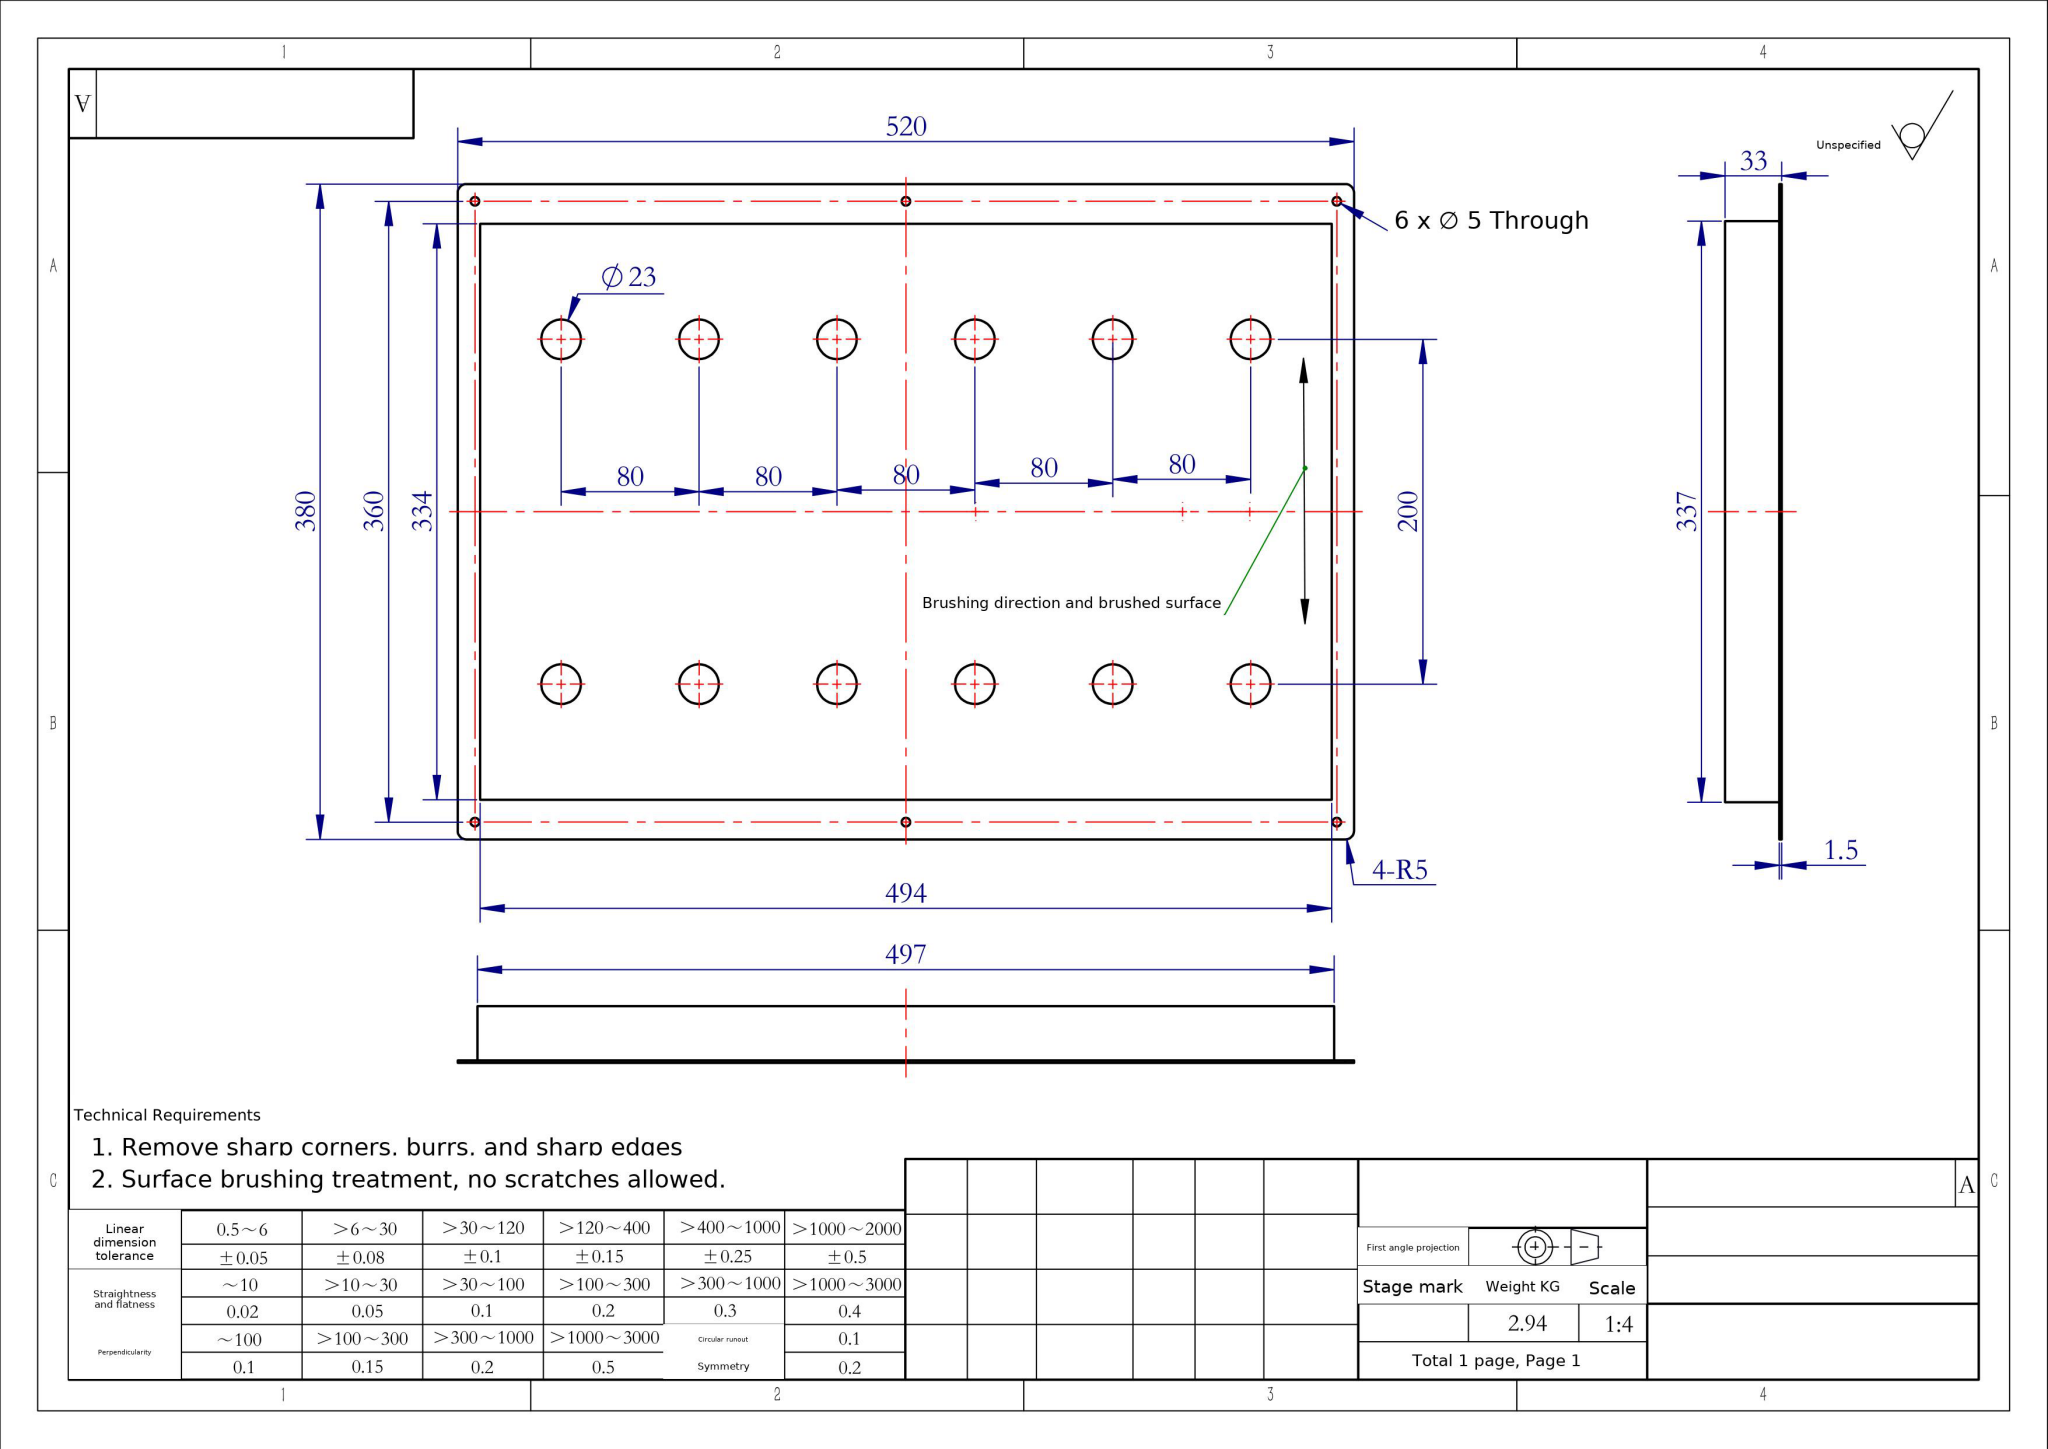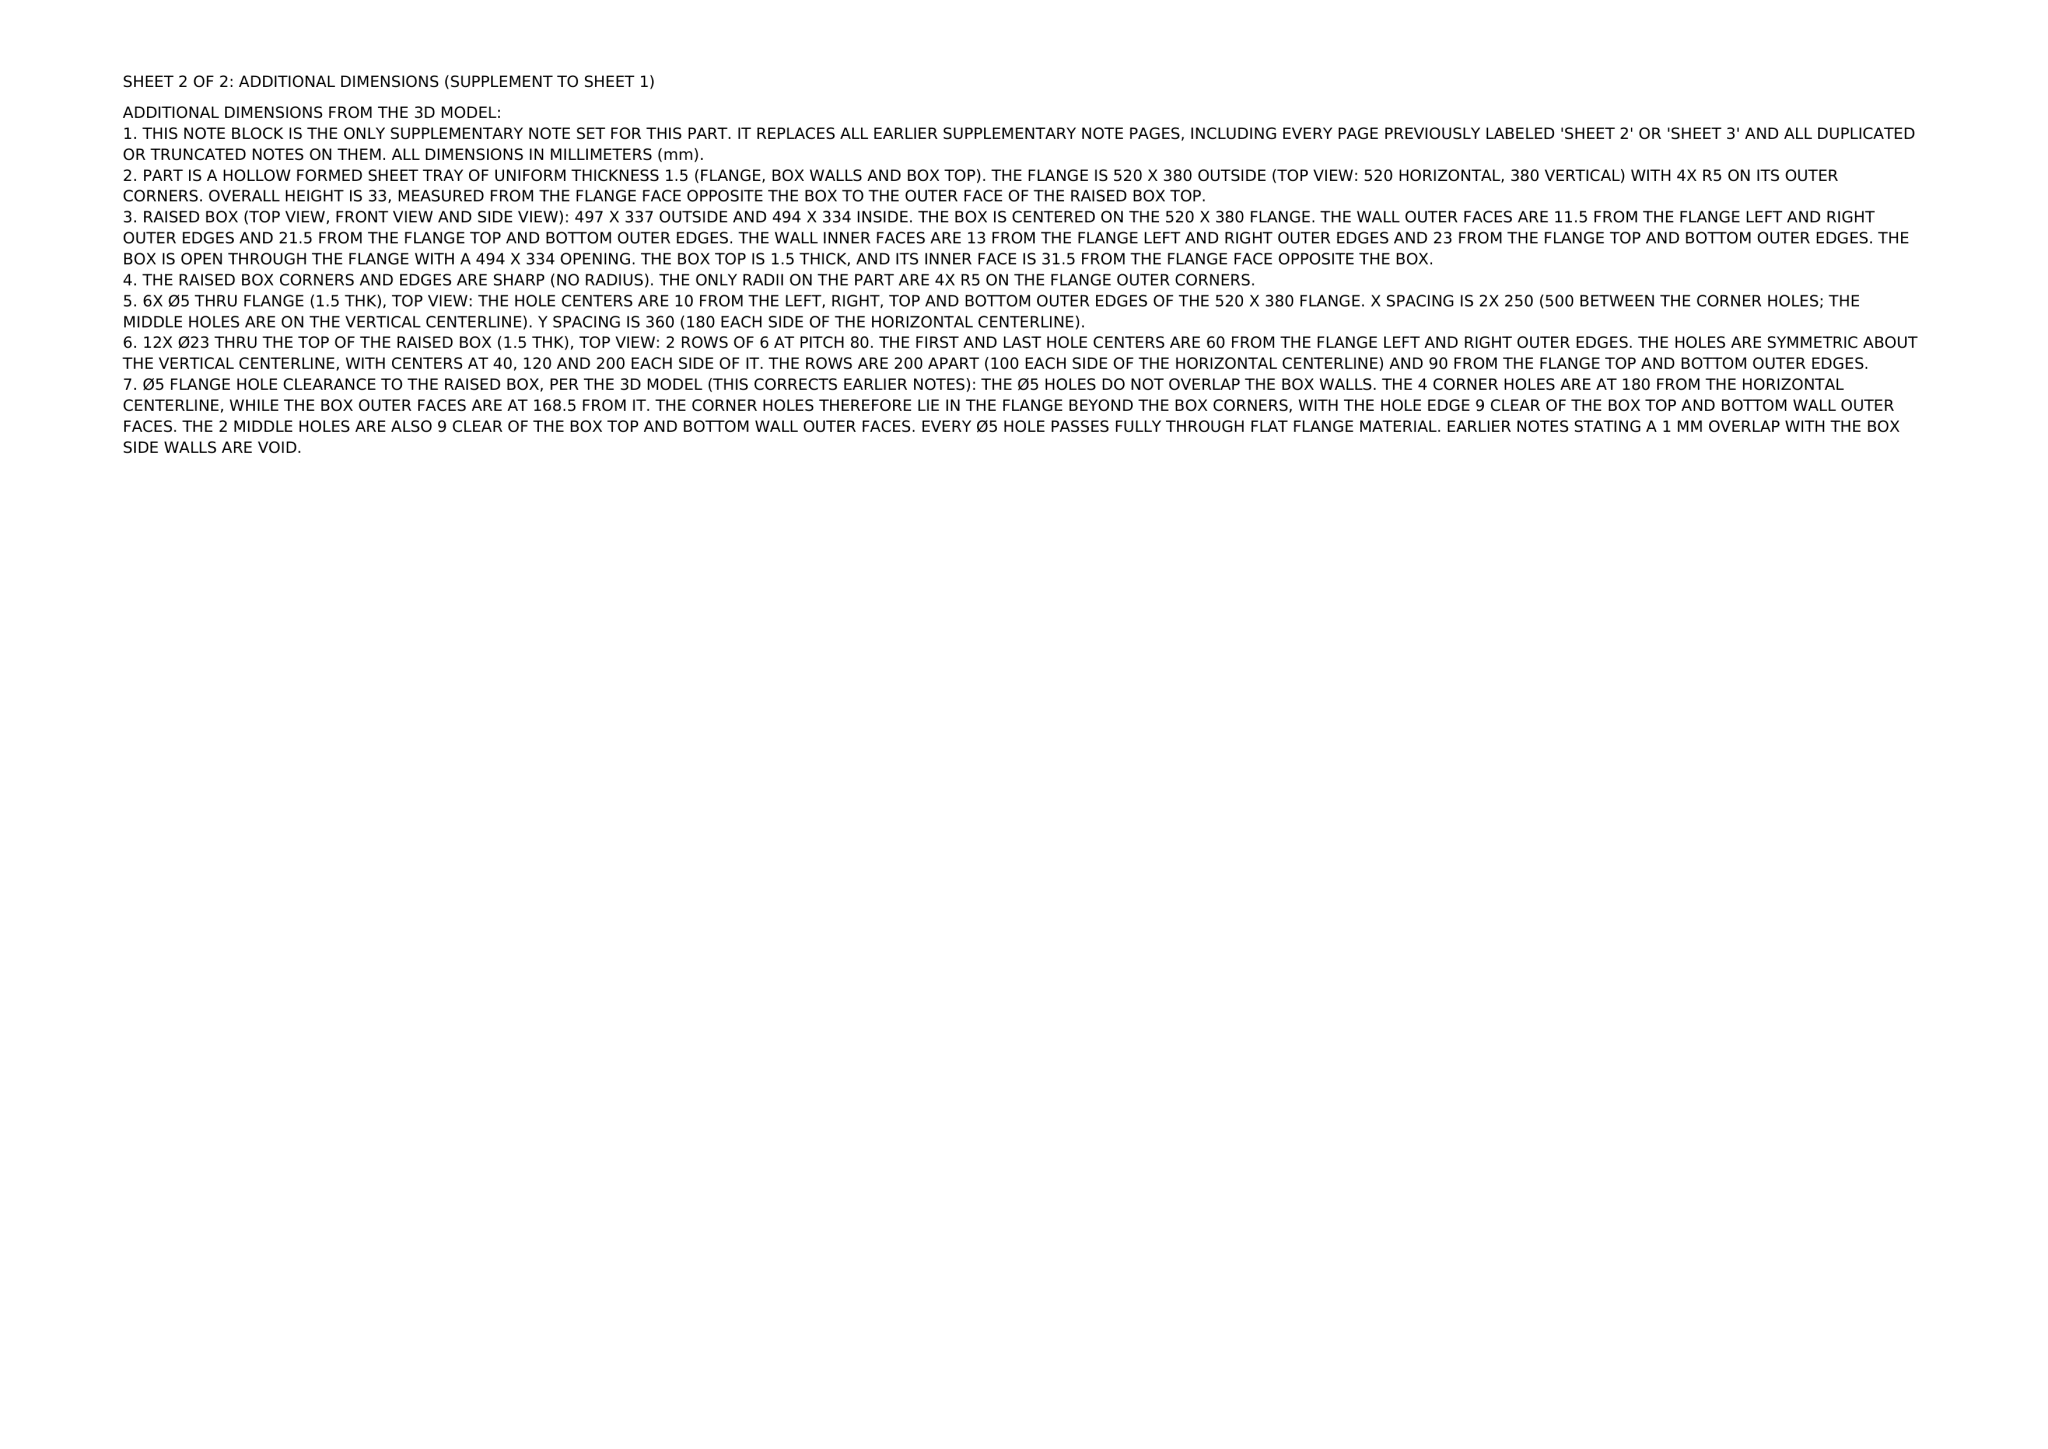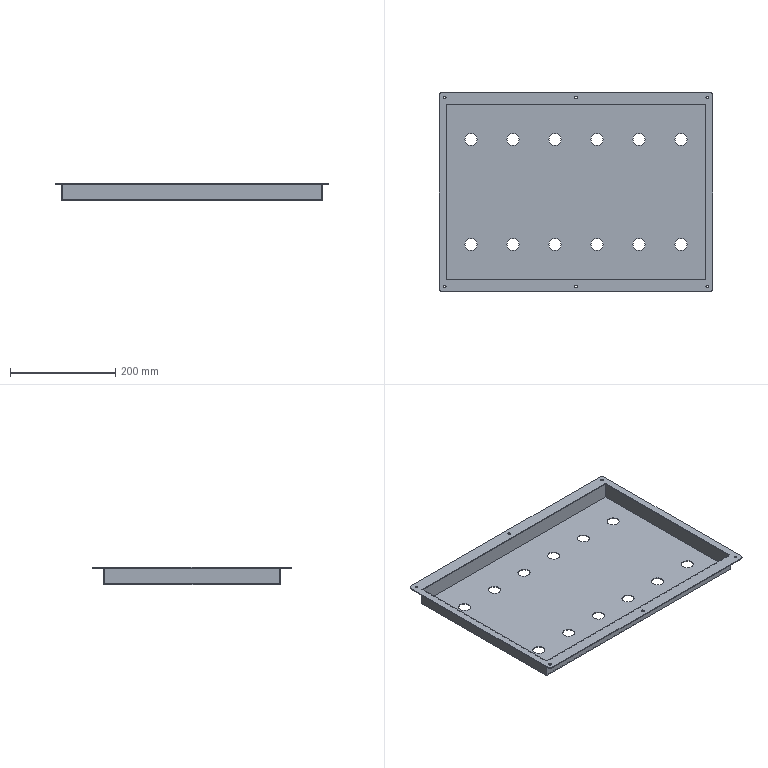Part | NX | mm | 1 solid | 60 faces | box 520 x 380 x 33 mm | volume 367242 mm3 | cylinder 40 | plane 20 | commonest cylinder face diameters 23 x24 5 x12 10 x4